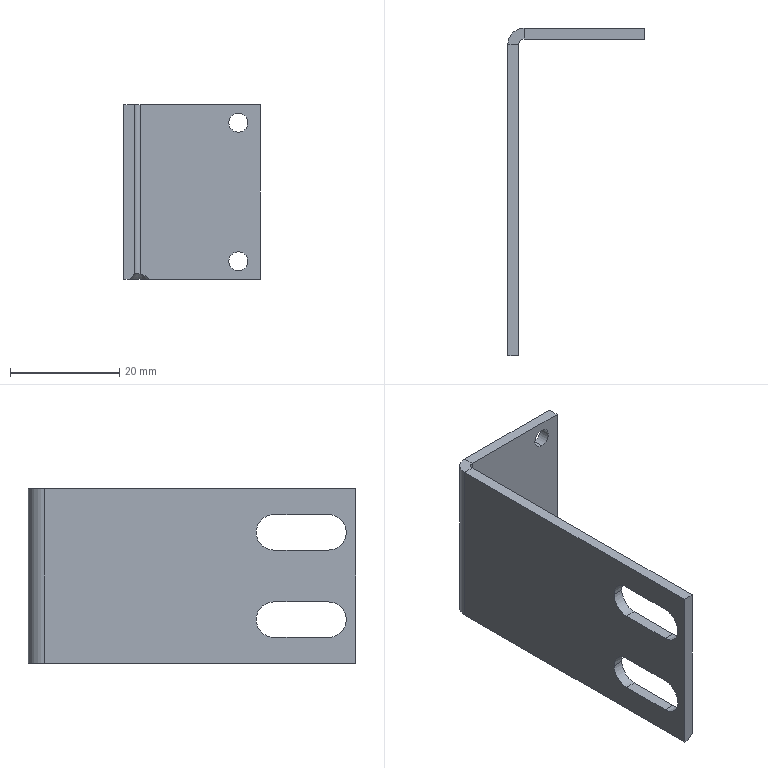Component | SolidWorks | 30-49A-1 | 1 solid | 30 faces | box 25 x 60 x 32 mm | volume 4796 mm3 | plane 17 | cylinder 12 | cone 1 | commonest cylinder face diameters 6.5 x6 3.5 x4 6 x1 2 x1
STEP:
#1=CARTESIAN_POINT('',(-33.473,1.02,11.797));
#2=VERTEX_POINT('',#1);
#3=CARTESIAN_POINT('',(-33.473,1.02,11.659));
#4=VERTEX_POINT('',#3);
#5=CARTESIAN_POINT('',(-33.473,1.02,11.728));
#6=DIRECTION('',(-0.,1.,-0.));
#7=DIRECTION('',(0.,0.,-1.));
#8=AXIS2_PLACEMENT_3D('',#5,#6,#7);
#9=CIRCLE('',#8,0.0689);
#10=EDGE_CURVE('',#2,#4,#9,.T.);
#11=ORIENTED_EDGE('',*,*,#10,.F.);
#12=CARTESIAN_POINT('',(-33.473,1.099,11.797));
#13=VERTEX_POINT('',#12);
#14=CARTESIAN_POINT('',(-33.473,1.099,11.797));
#15=DIRECTION('',(-0.,1.,-0.));
#16=VECTOR('',#15,39.37);
#17=LINE('',#14,#16);
#18=EDGE_CURVE('',#2,#13,#17,.T.);
#19=ORIENTED_EDGE('',*,*,#18,.T.);
#20=CARTESIAN_POINT('',(-33.473,1.099,11.659));
#21=VERTEX_POINT('',#20);
#22=CARTESIAN_POINT('',(-33.473,1.099,11.728));
#23=DIRECTION('',(-0.,1.,-0.));
#24=DIRECTION('',(0.,0.,-1.));
#25=AXIS2_PLACEMENT_3D('',#22,#23,#24);
#26=CIRCLE('',#25,0.0689);
#27=EDGE_CURVE('',#13,#21,#26,.T.);
#28=ORIENTED_EDGE('',*,*,#27,.T.);
#29=CARTESIAN_POINT('',(-33.473,1.099,11.659));
#30=DIRECTION('',(-0.,1.,-0.));
#31=VECTOR('',#30,39.37);
#32=LINE('',#29,#31);
#33=EDGE_CURVE('',#4,#21,#32,.T.);
#34=ORIENTED_EDGE('',*,*,#33,.F.);
#35=EDGE_LOOP('',(#11,#19,#28,#34));
#36=FACE_OUTER_BOUND('',#35,.T.);
#37=CARTESIAN_POINT('',(-33.473,1.099,11.728));
#38=DIRECTION('',(-0.,1.,-0.));
#39=DIRECTION('',(0.,0.,-1.));
#40=AXIS2_PLACEMENT_3D('',#37,#38,#39);
#41=CYLINDRICAL_SURFACE('',#40,0.0689);
#42=ADVANCED_FACE('',(#36),#41,.F.);
#43=CARTESIAN_POINT('',(-33.473,1.02,10.797));
#44=VERTEX_POINT('',#43);
#45=CARTESIAN_POINT('',(-33.473,1.02,10.659));
#46=VERTEX_POINT('',#45);
#47=CARTESIAN_POINT('',(-33.473,1.02,10.728));
#48=DIRECTION('',(-0.,1.,-0.));
#49=DIRECTION('',(0.,0.,-1.));
#50=AXIS2_PLACEMENT_3D('',#47,#48,#49);
#51=CIRCLE('',#50,0.0689);
#52=EDGE_CURVE('',#44,#46,#51,.T.);
#53=ORIENTED_EDGE('',*,*,#52,.F.);
#54=CARTESIAN_POINT('',(-33.473,1.099,10.797));
#55=VERTEX_POINT('',#54);
#56=CARTESIAN_POINT('',(-33.473,1.099,10.797));
#57=DIRECTION('',(-0.,1.,-0.));
#58=VECTOR('',#57,39.37);
#59=LINE('',#56,#58);
#60=EDGE_CURVE('',#44,#55,#59,.T.);
#61=ORIENTED_EDGE('',*,*,#60,.T.);
#62=CARTESIAN_POINT('',(-33.473,1.099,10.659));
#63=VERTEX_POINT('',#62);
#64=CARTESIAN_POINT('',(-33.473,1.099,10.728));
#65=DIRECTION('',(-0.,1.,-0.));
#66=DIRECTION('',(0.,0.,-1.));
#67=AXIS2_PLACEMENT_3D('',#64,#65,#66);
#68=CIRCLE('',#67,0.0689);
#69=EDGE_CURVE('',#55,#63,#68,.T.);
#70=ORIENTED_EDGE('',*,*,#69,.T.);
#71=CARTESIAN_POINT('',(-33.473,1.099,10.659));
#72=DIRECTION('',(-0.,1.,-0.));
#73=VECTOR('',#72,39.37);
#74=LINE('',#71,#73);
#75=EDGE_CURVE('',#46,#63,#74,.T.);
#76=ORIENTED_EDGE('',*,*,#75,.F.);
#77=EDGE_LOOP('',(#53,#61,#70,#76));
#78=FACE_OUTER_BOUND('',#77,.T.);
#79=CARTESIAN_POINT('',(-33.473,1.099,10.728));
#80=DIRECTION('',(-0.,1.,-0.));
#81=DIRECTION('',(0.,0.,-1.));
#82=AXIS2_PLACEMENT_3D('',#79,#80,#81);
#83=CYLINDRICAL_SURFACE('',#82,0.0689);
#84=ADVANCED_FACE('',(#78),#83,.F.);
#85=CARTESIAN_POINT('',(-34.221,-0.5449,11.543));
#86=VERTEX_POINT('',#85);
#87=CARTESIAN_POINT('',(-34.221,-0.6729,11.415));
#88=VERTEX_POINT('',#87);
#89=CARTESIAN_POINT('',(-34.221,-0.6729,11.543));
#90=DIRECTION('',(-1.,-0.,0.));
#91=DIRECTION('',(0.,1.,0.));
#92=AXIS2_PLACEMENT_3D('',#89,#90,#91);
#93=CIRCLE('',#92,0.128);
#94=EDGE_CURVE('',#86,#88,#93,.T.);
#95=ORIENTED_EDGE('',*,*,#94,.F.);
#96=CARTESIAN_POINT('',(-34.3,-0.5449,11.543));
#97=VERTEX_POINT('',#96);
#98=CARTESIAN_POINT('',(-33.315,-0.5449,11.543));
#99=DIRECTION('',(-1.,-0.,0.));
#100=VECTOR('',#99,39.37);
#101=LINE('',#98,#100);
#102=EDGE_CURVE('',#86,#97,#101,.T.);
#103=ORIENTED_EDGE('',*,*,#102,.T.);
#104=CARTESIAN_POINT('',(-34.3,-0.6729,11.415));
#105=VERTEX_POINT('',#104);
#106=CARTESIAN_POINT('',(-34.3,-0.6729,11.543));
#107=DIRECTION('',(-1.,-0.,0.));
#108=DIRECTION('',(0.,1.,0.));
#109=AXIS2_PLACEMENT_3D('',#106,#107,#108);
#110=CIRCLE('',#109,0.128);
#111=EDGE_CURVE('',#97,#105,#110,.T.);
#112=ORIENTED_EDGE('',*,*,#111,.T.);
#113=CARTESIAN_POINT('',(-33.315,-0.6729,11.415));
#114=DIRECTION('',(-1.,-0.,0.));
#115=VECTOR('',#114,39.37);
#116=LINE('',#113,#115);
#117=EDGE_CURVE('',#88,#105,#116,.T.);
#118=ORIENTED_EDGE('',*,*,#117,.F.);
#119=EDGE_LOOP('',(#95,#103,#112,#118));
#120=FACE_OUTER_BOUND('',#119,.T.);
#121=CARTESIAN_POINT('',(-33.315,-0.6729,11.543));
#122=DIRECTION('',(-1.,-0.,0.));
#123=DIRECTION('',(0.,1.,0.));
#124=AXIS2_PLACEMENT_3D('',#121,#122,#123);
#125=CYLINDRICAL_SURFACE('',#124,0.128);
#126=ADVANCED_FACE('',(#120),#125,.F.);
#127=CARTESIAN_POINT('',(-34.221,-0.5449,10.913));
#128=VERTEX_POINT('',#127);
#129=CARTESIAN_POINT('',(-34.221,-0.6729,10.785));
#130=VERTEX_POINT('',#129);
#131=CARTESIAN_POINT('',(-34.221,-0.6729,10.913));
#132=DIRECTION('',(-1.,-0.,0.));
#133=DIRECTION('',(0.,1.,0.));
#134=AXIS2_PLACEMENT_3D('',#131,#132,#133);
#135=CIRCLE('',#134,0.128);
#136=EDGE_CURVE('',#128,#130,#135,.T.);
#137=ORIENTED_EDGE('',*,*,#136,.F.);
#138=CARTESIAN_POINT('',(-34.3,-0.5449,10.913));
#139=VERTEX_POINT('',#138);
#140=CARTESIAN_POINT('',(-33.315,-0.5449,10.913));
#141=DIRECTION('',(-1.,-0.,0.));
#142=VECTOR('',#141,39.37);
#143=LINE('',#140,#142);
#144=EDGE_CURVE('',#128,#139,#143,.T.);
#145=ORIENTED_EDGE('',*,*,#144,.T.);
#146=CARTESIAN_POINT('',(-34.3,-0.6729,10.785));
#147=VERTEX_POINT('',#146);
#148=CARTESIAN_POINT('',(-34.3,-0.6729,10.913));
#149=DIRECTION('',(-1.,-0.,0.));
#150=DIRECTION('',(0.,-1.,0.));
#151=AXIS2_PLACEMENT_3D('',#148,#149,#150);
#152=CIRCLE('',#151,0.128);
#153=EDGE_CURVE('',#139,#147,#152,.T.);
#154=ORIENTED_EDGE('',*,*,#153,.T.);
#155=CARTESIAN_POINT('',(-33.315,-0.6729,10.785));
#156=DIRECTION('',(-1.,-0.,0.));
#157=VECTOR('',#156,39.37);
#158=LINE('',#155,#157);
#159=EDGE_CURVE('',#130,#147,#158,.T.);
#160=ORIENTED_EDGE('',*,*,#159,.F.);
#161=EDGE_LOOP('',(#137,#145,#154,#160));
#162=FACE_OUTER_BOUND('',#161,.T.);
#163=CARTESIAN_POINT('',(-33.315,-0.6729,10.913));
#164=DIRECTION('',(-1.,-0.,0.));
#165=DIRECTION('',(0.,1.,0.));
#166=AXIS2_PLACEMENT_3D('',#163,#164,#165);
#167=CYLINDRICAL_SURFACE('',#166,0.128);
#168=ADVANCED_FACE('',(#162),#167,.F.);
#169=CARTESIAN_POINT('',(-34.181,1.059,10.598));
#170=VERTEX_POINT('',#169);
#171=CARTESIAN_POINT('',(-34.181,1.099,10.598));
#172=VERTEX_POINT('',#171);
#173=CARTESIAN_POINT('',(-34.181,1.02,10.598));
#174=DIRECTION('',(-0.,1.,-0.));
#175=VECTOR('',#174,39.37);
#176=LINE('',#173,#175);
#177=EDGE_CURVE('',#170,#172,#176,.T.);
#178=ORIENTED_EDGE('',*,*,#177,.F.);
#179=CARTESIAN_POINT('',(-34.26,0.9806,10.598));
#180=VERTEX_POINT('',#179);
#181=CARTESIAN_POINT('',(-34.181,0.9806,10.598));
#182=DIRECTION('',(0.,0.,1.));
#183=DIRECTION('',(-1.,-0.,0.));
#184=AXIS2_PLACEMENT_3D('',#181,#182,#183);
#185=CIRCLE('',#184,0.07874);
#186=EDGE_CURVE('',#170,#180,#185,.T.);
#187=ORIENTED_EDGE('',*,*,#186,.T.);
#188=CARTESIAN_POINT('',(-34.3,0.9806,10.598));
#189=VERTEX_POINT('',#188);
#190=CARTESIAN_POINT('',(-34.3,0.9806,10.598));
#191=DIRECTION('',(1.,0.,-0.));
#192=VECTOR('',#191,39.37);
#193=LINE('',#190,#192);
#194=EDGE_CURVE('',#189,#180,#193,.T.);
#195=ORIENTED_EDGE('',*,*,#194,.F.);
#196=CARTESIAN_POINT('',(-34.181,0.9806,10.598));
#197=DIRECTION('',(0.,0.,1.));
#198=DIRECTION('',(-1.,-0.,0.));
#199=AXIS2_PLACEMENT_3D('',#196,#197,#198);
#200=CIRCLE('',#199,0.1181);
#201=EDGE_CURVE('',#172,#189,#200,.T.);
#202=ORIENTED_EDGE('',*,*,#201,.F.);
#203=EDGE_LOOP('',(#178,#187,#195,#202));
#204=FACE_OUTER_BOUND('',#203,.T.);
#205=CARTESIAN_POINT('',(-34.3,0.9806,10.598));
#206=DIRECTION('',(-0.,-0.,-1.));
#207=DIRECTION('',(-1.,-0.,0.));
#208=AXIS2_PLACEMENT_3D('',#205,#206,#207);
#209=PLANE('',#208);
#210=ADVANCED_FACE('',(#204),#209,.T.);
#211=ORIENTED_EDGE('',*,*,#194,.T.);
#212=CARTESIAN_POINT('',(-34.26,-1.263,10.598));
#213=VERTEX_POINT('',#212);
#214=CARTESIAN_POINT('',(-34.26,-1.263,10.598));
#215=DIRECTION('',(0.,-1.,0.));
#216=VECTOR('',#215,39.37);
#217=LINE('',#214,#216);
#218=EDGE_CURVE('',#180,#213,#217,.T.);
#219=ORIENTED_EDGE('',*,*,#218,.T.);
#220=CARTESIAN_POINT('',(-34.3,-1.263,10.598));
#221=VERTEX_POINT('',#220);
#222=CARTESIAN_POINT('',(-34.3,-1.263,10.598));
#223=DIRECTION('',(1.,0.,-0.));
#224=VECTOR('',#223,39.37);
#225=LINE('',#222,#224);
#226=EDGE_CURVE('',#221,#213,#225,.T.);
#227=ORIENTED_EDGE('',*,*,#226,.F.);
#228=CARTESIAN_POINT('',(-34.3,1.099,10.598));
#229=DIRECTION('',(0.,-1.,0.));
#230=VECTOR('',#229,39.37);
#231=LINE('',#228,#230);
#232=EDGE_CURVE('',#189,#221,#231,.T.);
#233=ORIENTED_EDGE('',*,*,#232,.F.);
#234=EDGE_LOOP('',(#211,#219,#227,#233));
#235=FACE_OUTER_BOUND('',#234,.T.);
#236=CARTESIAN_POINT('',(-34.181,1.02,10.598));
#237=DIRECTION('',(-0.,-0.,-1.));
#238=DIRECTION('',(-1.,-0.,0.));
#239=AXIS2_PLACEMENT_3D('',#236,#237,#238);
#240=PLANE('',#239);
#241=ADVANCED_FACE('',(#235),#240,.T.);
#242=CARTESIAN_POINT('',(-34.181,1.099,11.858));
#243=VERTEX_POINT('',#242);
#244=CARTESIAN_POINT('',(-34.181,1.02,11.858));
#245=VERTEX_POINT('',#244);
#246=CARTESIAN_POINT('',(-34.181,1.099,11.858));
#247=DIRECTION('',(0.,-1.,0.));
#248=VECTOR('',#247,39.37);
#249=LINE('',#246,#248);
#250=EDGE_CURVE('',#243,#245,#249,.T.);
#251=ORIENTED_EDGE('',*,*,#250,.F.);
#252=CARTESIAN_POINT('',(-34.3,0.9806,11.858));
#253=VERTEX_POINT('',#252);
#254=CARTESIAN_POINT('',(-34.181,0.9806,11.858));
#255=DIRECTION('',(0.,0.,1.));
#256=DIRECTION('',(-1.,-0.,0.));
#257=AXIS2_PLACEMENT_3D('',#254,#255,#256);
#258=CIRCLE('',#257,0.1181);
#259=EDGE_CURVE('',#243,#253,#258,.T.);
#260=ORIENTED_EDGE('',*,*,#259,.T.);
#261=CARTESIAN_POINT('',(-34.221,0.9806,11.858));
#262=VERTEX_POINT('',#261);
#263=CARTESIAN_POINT('',(-34.221,0.9806,11.858));
#264=DIRECTION('',(-1.,-0.,0.));
#265=VECTOR('',#264,39.37);
#266=LINE('',#263,#265);
#267=EDGE_CURVE('',#262,#253,#266,.T.);
#268=ORIENTED_EDGE('',*,*,#267,.F.);
#269=CARTESIAN_POINT('',(-34.181,0.9806,11.858));
#270=DIRECTION('',(0.,0.,1.));
#271=DIRECTION('',(-1.,-0.,0.));
#272=AXIS2_PLACEMENT_3D('',#269,#270,#271);
#273=CIRCLE('',#272,0.03937);
#274=EDGE_CURVE('',#245,#262,#273,.T.);
#275=ORIENTED_EDGE('',*,*,#274,.F.);
#276=EDGE_LOOP('',(#251,#260,#268,#275));
#277=FACE_OUTER_BOUND('',#276,.T.);
#278=CARTESIAN_POINT('',(-34.181,1.099,11.858));
#279=DIRECTION('',(0.,0.,1.));
#280=DIRECTION('',(1.,0.,-0.));
#281=AXIS2_PLACEMENT_3D('',#278,#279,#280);
#282=PLANE('',#281);
#283=ADVANCED_FACE('',(#277),#282,.T.);
#284=CARTESIAN_POINT('',(-33.315,1.099,11.858));
#285=VERTEX_POINT('',#284);
#286=CARTESIAN_POINT('',(-33.315,1.099,11.858));
#287=DIRECTION('',(-1.,-0.,0.));
#288=VECTOR('',#287,39.37);
#289=LINE('',#286,#288);
#290=EDGE_CURVE('',#285,#243,#289,.T.);
#291=ORIENTED_EDGE('',*,*,#290,.T.);
#292=ORIENTED_EDGE('',*,*,#250,.T.);
#293=CARTESIAN_POINT('',(-33.315,1.02,11.858));
#294=VERTEX_POINT('',#293);
#295=CARTESIAN_POINT('',(-33.315,1.02,11.858));
#296=DIRECTION('',(-1.,-0.,0.));
#297=VECTOR('',#296,39.37);
#298=LINE('',#295,#297);
#299=EDGE_CURVE('',#294,#245,#298,.T.);
#300=ORIENTED_EDGE('',*,*,#299,.F.);
#301=CARTESIAN_POINT('',(-33.315,1.02,11.858));
#302=DIRECTION('',(-0.,1.,-0.));
#303=VECTOR('',#302,39.37);
#304=LINE('',#301,#303);
#305=EDGE_CURVE('',#294,#285,#304,.T.);
#306=ORIENTED_EDGE('',*,*,#305,.T.);
#307=EDGE_LOOP('',(#291,#292,#300,#306));
#308=FACE_OUTER_BOUND('',#307,.T.);
#309=CARTESIAN_POINT('',(-34.221,0.9806,11.858));
#310=DIRECTION('',(0.,0.,1.));
#311=DIRECTION('',(1.,0.,-0.));
#312=AXIS2_PLACEMENT_3D('',#309,#310,#311);
#313=PLANE('',#312);
#314=ADVANCED_FACE('',(#308),#313,.T.);
#315=CARTESIAN_POINT('',(-34.221,-1.067,11.415));
#316=VERTEX_POINT('',#315);
#317=CARTESIAN_POINT('',(-34.221,1.099,11.415));
#318=DIRECTION('',(0.,-1.,0.));
#319=VECTOR('',#318,39.37);
#320=LINE('',#317,#319);
#321=EDGE_CURVE('',#88,#316,#320,.T.);
#322=ORIENTED_EDGE('',*,*,#321,.T.);
#323=CARTESIAN_POINT('',(-34.221,-1.067,11.671));
#324=VERTEX_POINT('',#323);
#325=CARTESIAN_POINT('',(-34.221,-1.067,11.543));
#326=DIRECTION('',(-1.,-0.,0.));
#327=DIRECTION('',(0.,1.,0.));
#328=AXIS2_PLACEMENT_3D('',#325,#326,#327);
#329=CIRCLE('',#328,0.128);
#330=EDGE_CURVE('',#316,#324,#329,.T.);
#331=ORIENTED_EDGE('',*,*,#330,.T.);
#332=CARTESIAN_POINT('',(-34.221,-0.6729,11.671));
#333=VERTEX_POINT('',#332);
#334=CARTESIAN_POINT('',(-34.221,1.099,11.671));
#335=DIRECTION('',(-0.,1.,-0.));
#336=VECTOR('',#335,39.37);
#337=LINE('',#334,#336);
#338=EDGE_CURVE('',#324,#333,#337,.T.);
#339=ORIENTED_EDGE('',*,*,#338,.T.);
#340=CARTESIAN_POINT('',(-34.221,-0.6729,11.543));
#341=DIRECTION('',(-1.,-0.,0.));
#342=DIRECTION('',(0.,1.,0.));
#343=AXIS2_PLACEMENT_3D('',#340,#341,#342);
#344=CIRCLE('',#343,0.128);
#345=EDGE_CURVE('',#333,#86,#344,.T.);
#346=ORIENTED_EDGE('',*,*,#345,.T.);
#347=ORIENTED_EDGE('',*,*,#94,.T.);
#348=EDGE_LOOP('',(#322,#331,#339,#346,#347));
#349=FACE_BOUND('',#348,.T.);
#350=CARTESIAN_POINT('',(-34.221,-1.067,11.041));
#351=VERTEX_POINT('',#350);
#352=CARTESIAN_POINT('',(-34.221,-0.6729,11.041));
#353=VERTEX_POINT('',#352);
#354=CARTESIAN_POINT('',(-34.221,1.099,11.041));
#355=DIRECTION('',(-0.,1.,-0.));
#356=VECTOR('',#355,39.37);
#357=LINE('',#354,#356);
#358=EDGE_CURVE('',#351,#353,#357,.T.);
#359=ORIENTED_EDGE('',*,*,#358,.T.);
#360=CARTESIAN_POINT('',(-34.221,-0.6729,10.913));
#361=DIRECTION('',(-1.,-0.,0.));
#362=DIRECTION('',(0.,1.,0.));
#363=AXIS2_PLACEMENT_3D('',#360,#361,#362);
#364=CIRCLE('',#363,0.128);
#365=EDGE_CURVE('',#353,#128,#364,.T.);
#366=ORIENTED_EDGE('',*,*,#365,.T.);
#367=ORIENTED_EDGE('',*,*,#136,.T.);
#368=CARTESIAN_POINT('',(-34.221,-1.067,10.785));
#369=VERTEX_POINT('',#368);
#370=CARTESIAN_POINT('',(-34.221,1.099,10.785));
#371=DIRECTION('',(0.,-1.,0.));
#372=VECTOR('',#371,39.37);
#373=LINE('',#370,#372);
#374=EDGE_CURVE('',#130,#369,#373,.T.);
#375=ORIENTED_EDGE('',*,*,#374,.T.);
#376=CARTESIAN_POINT('',(-34.221,-1.067,10.913));
#377=DIRECTION('',(-1.,-0.,0.));
#378=DIRECTION('',(0.,1.,0.));
#379=AXIS2_PLACEMENT_3D('',#376,#377,#378);
#380=CIRCLE('',#379,0.128);
#381=EDGE_CURVE('',#369,#351,#380,.T.);
#382=ORIENTED_EDGE('',*,*,#381,.T.);
#383=EDGE_LOOP('',(#359,#366,#367,#375,#382));
#384=FACE_BOUND('',#383,.T.);
#385=CARTESIAN_POINT('',(-34.221,-1.263,10.637));
#386=VERTEX_POINT('',#385);
#387=CARTESIAN_POINT('',(-34.221,-1.263,11.858));
#388=VERTEX_POINT('',#387);
#389=CARTESIAN_POINT('',(-34.221,-1.263,10.598));
#390=DIRECTION('',(0.,0.,1.));
#391=VECTOR('',#390,39.37);
#392=LINE('',#389,#391);
#393=EDGE_CURVE('',#386,#388,#392,.T.);
#394=ORIENTED_EDGE('',*,*,#393,.F.);
#395=CARTESIAN_POINT('',(-34.221,0.9806,10.637));
#396=VERTEX_POINT('',#395);
#397=CARTESIAN_POINT('',(-34.221,0.9806,10.637));
#398=DIRECTION('',(-0.,1.,-0.));
#399=VECTOR('',#398,39.37);
#400=LINE('',#397,#399);
#401=EDGE_CURVE('',#386,#396,#400,.T.);
#402=ORIENTED_EDGE('',*,*,#401,.T.);
#403=CARTESIAN_POINT('',(-34.221,0.9806,10.598));
#404=DIRECTION('',(0.,0.,1.));
#405=VECTOR('',#404,39.37);
#406=LINE('',#403,#405);
#407=EDGE_CURVE('',#396,#262,#406,.T.);
#408=ORIENTED_EDGE('',*,*,#407,.T.);
#409=CARTESIAN_POINT('',(-34.221,1.099,11.858));
#410=DIRECTION('',(0.,-1.,0.));
#411=VECTOR('',#410,39.37);
#412=LINE('',#409,#411);
#413=EDGE_CURVE('',#262,#388,#412,.T.);
#414=ORIENTED_EDGE('',*,*,#413,.T.);
#415=EDGE_LOOP('',(#394,#402,#408,#414));
#416=FACE_OUTER_BOUND('',#415,.T.);
#417=CARTESIAN_POINT('',(-34.221,1.099,10.598));
#418=DIRECTION('',(-1.,-0.,0.));
#419=DIRECTION('',(-0.,1.,-0.));
#420=AXIS2_PLACEMENT_3D('',#417,#418,#419);
#421=PLANE('',#420);
#422=ADVANCED_FACE('',(#349,#384,#416),#421,.F.);
#423=ORIENTED_EDGE('',*,*,#226,.T.);
#424=CARTESIAN_POINT('',(-34.28,-1.263,10.578));
#425=DIRECTION('',(0.7071,0.,0.7071));
#426=VECTOR('',#425,39.37);
#427=LINE('',#424,#426);
#428=EDGE_CURVE('',#213,#386,#427,.T.);
#429=ORIENTED_EDGE('',*,*,#428,.T.);
#430=ORIENTED_EDGE('',*,*,#393,.T.);
#431=CARTESIAN_POINT('',(-34.3,-1.263,11.858));
#432=VERTEX_POINT('',#431);
#433=CARTESIAN_POINT('',(-34.3,-1.263,11.858));
#434=DIRECTION('',(1.,0.,-0.));
#435=VECTOR('',#434,39.37);
#436=LINE('',#433,#435);
#437=EDGE_CURVE('',#432,#388,#436,.T.);
#438=ORIENTED_EDGE('',*,*,#437,.F.);
#439=CARTESIAN_POINT('',(-34.3,-1.263,10.598));
#440=DIRECTION('',(0.,0.,1.));
#441=VECTOR('',#440,39.37);
#442=LINE('',#439,#441);
#443=EDGE_CURVE('',#221,#432,#442,.T.);
#444=ORIENTED_EDGE('',*,*,#443,.F.);
#445=EDGE_LOOP('',(#423,#429,#430,#438,#444));
#446=FACE_OUTER_BOUND('',#445,.T.);
#447=CARTESIAN_POINT('',(-34.3,-1.263,10.598));
#448=DIRECTION('',(0.,-1.,0.));
#449=DIRECTION('',(0.,0.,1.));
#450=AXIS2_PLACEMENT_3D('',#447,#448,#449);
#451=PLANE('',#450);
#452=ADVANCED_FACE('',(#446),#451,.T.);
#453=CARTESIAN_POINT('',(-34.3,-1.067,11.415));
#454=VERTEX_POINT('',#453);
#455=CARTESIAN_POINT('',(-34.3,-1.067,11.671));
#456=VERTEX_POINT('',#455);
#457=CARTESIAN_POINT('',(-34.3,-1.067,11.543));
#458=DIRECTION('',(-1.,-0.,0.));
#459=DIRECTION('',(0.,-1.,0.));
#460=AXIS2_PLACEMENT_3D('',#457,#458,#459);
#461=CIRCLE('',#460,0.128);
#462=EDGE_CURVE('',#454,#456,#461,.T.);
#463=ORIENTED_EDGE('',*,*,#462,.F.);
#464=CARTESIAN_POINT('',(-34.3,-0.6729,11.415));
#465=DIRECTION('',(0.,-1.,0.));
#466=VECTOR('',#465,39.37);
#467=LINE('',#464,#466);
#468=EDGE_CURVE('',#105,#454,#467,.T.);
#469=ORIENTED_EDGE('',*,*,#468,.F.);
#470=ORIENTED_EDGE('',*,*,#111,.F.);
#471=CARTESIAN_POINT('',(-34.3,-0.6729,11.671));
#472=VERTEX_POINT('',#471);
#473=CARTESIAN_POINT('',(-34.3,-0.6729,11.543));
#474=DIRECTION('',(-1.,-0.,0.));
#475=DIRECTION('',(0.,1.,0.));
#476=AXIS2_PLACEMENT_3D('',#473,#474,#475);
#477=CIRCLE('',#476,0.128);
#478=EDGE_CURVE('',#472,#97,#477,.T.);
#479=ORIENTED_EDGE('',*,*,#478,.F.);
#480=CARTESIAN_POINT('',(-34.3,-0.6729,11.671));
#481=DIRECTION('',(-0.,1.,-0.));
#482=VECTOR('',#481,39.37);
#483=LINE('',#480,#482);
#484=EDGE_CURVE('',#456,#472,#483,.T.);
#485=ORIENTED_EDGE('',*,*,#484,.F.);
#486=EDGE_LOOP('',(#463,#469,#470,#479,#485));
#487=FACE_BOUND('',#486,.T.);
#488=CARTESIAN_POINT('',(-34.3,-0.6729,11.041));
#489=VERTEX_POINT('',#488);
#490=CARTESIAN_POINT('',(-34.3,-0.6729,10.913));
#491=DIRECTION('',(-1.,-0.,0.));
#492=DIRECTION('',(0.,-1.,0.));
#493=AXIS2_PLACEMENT_3D('',#490,#491,#492);
#494=CIRCLE('',#493,0.128);
#495=EDGE_CURVE('',#489,#139,#494,.T.);
#496=ORIENTED_EDGE('',*,*,#495,.F.);
#497=CARTESIAN_POINT('',(-34.3,-1.067,11.041));
#498=VERTEX_POINT('',#497);
#499=CARTESIAN_POINT('',(-34.3,-0.6729,11.041));
#500=DIRECTION('',(-0.,1.,-0.));
#501=VECTOR('',#500,39.37);
#502=LINE('',#499,#501);
#503=EDGE_CURVE('',#498,#489,#502,.T.);
#504=ORIENTED_EDGE('',*,*,#503,.F.);
#505=CARTESIAN_POINT('',(-34.3,-1.067,10.785));
#506=VERTEX_POINT('',#505);
#507=CARTESIAN_POINT('',(-34.3,-1.067,10.913));
#508=DIRECTION('',(-1.,-0.,0.));
#509=DIRECTION('',(0.,1.,0.));
#510=AXIS2_PLACEMENT_3D('',#507,#508,#509);
#511=CIRCLE('',#510,0.128);
#512=EDGE_CURVE('',#506,#498,#511,.T.);
#513=ORIENTED_EDGE('',*,*,#512,.F.);
#514=CARTESIAN_POINT('',(-34.3,-0.6729,10.785));
#515=DIRECTION('',(0.,-1.,0.));
#516=VECTOR('',#515,39.37);
#517=LINE('',#514,#516);
#518=EDGE_CURVE('',#147,#506,#517,.T.);
#519=ORIENTED_EDGE('',*,*,#518,.F.);
#520=ORIENTED_EDGE('',*,*,#153,.F.);
#521=EDGE_LOOP('',(#496,#504,#513,#519,#520));
#522=FACE_BOUND('',#521,.T.);
#523=CARTESIAN_POINT('',(-34.3,1.099,11.858));
#524=DIRECTION('',(0.,-1.,0.));
#525=VECTOR('',#524,39.37);
#526=LINE('',#523,#525);
#527=EDGE_CURVE('',#253,#432,#526,.T.);
#528=ORIENTED_EDGE('',*,*,#527,.F.);
#529=CARTESIAN_POINT('',(-34.3,0.9806,10.598));
#530=DIRECTION('',(0.,0.,1.));
#531=VECTOR('',#530,39.37);
#532=LINE('',#529,#531);
#533=EDGE_CURVE('',#189,#253,#532,.T.);
#534=ORIENTED_EDGE('',*,*,#533,.F.);
#535=ORIENTED_EDGE('',*,*,#232,.T.);
#536=ORIENTED_EDGE('',*,*,#443,.T.);
#537=EDGE_LOOP('',(#528,#534,#535,#536));
#538=FACE_OUTER_BOUND('',#537,.T.);
#539=CARTESIAN_POINT('',(-34.3,1.099,10.598));
#540=DIRECTION('',(-1.,-0.,0.));
#541=DIRECTION('',(-0.,1.,-0.));
#542=AXIS2_PLACEMENT_3D('',#539,#540,#541);
#543=PLANE('',#542);
#544=ADVANCED_FACE('',(#487,#522,#538),#543,.T.);
#545=ORIENTED_EDGE('',*,*,#259,.F.);
#546=CARTESIAN_POINT('',(-34.181,1.099,10.598));
#547=DIRECTION('',(0.,0.,1.));
#548=VECTOR('',#547,39.37);
#549=LINE('',#546,#548);
#550=EDGE_CURVE('',#172,#243,#549,.T.);
#551=ORIENTED_EDGE('',*,*,#550,.F.);
#552=ORIENTED_EDGE('',*,*,#201,.T.);
#553=ORIENTED_EDGE('',*,*,#533,.T.);
#554=EDGE_LOOP('',(#545,#551,#552,#553));
#555=FACE_OUTER_BOUND('',#554,.T.);
#556=CARTESIAN_POINT('',(-34.181,0.9806,10.598));
#557=DIRECTION('',(0.,0.,1.));
#558=DIRECTION('',(1.,0.,0.));
#559=AXIS2_PLACEMENT_3D('',#556,#557,#558);
#560=CYLINDRICAL_SURFACE('',#559,0.1181);
#561=ADVANCED_FACE('',(#555),#560,.T.);
#562=CARTESIAN_POINT('',(-33.473,1.099,11.728));
#563=DIRECTION('',(-0.,1.,-0.));
#564=DIRECTION('',(0.,0.,-1.));
#565=AXIS2_PLACEMENT_3D('',#562,#563,#564);
#566=CIRCLE('',#565,0.0689);
#567=EDGE_CURVE('',#21,#13,#566,.T.);
#568=ORIENTED_EDGE('',*,*,#567,.F.);
#569=ORIENTED_EDGE('',*,*,#27,.F.);
#570=EDGE_LOOP('',(#568,#569));
#571=FACE_BOUND('',#570,.T.);
#572=CARTESIAN_POINT('',(-33.473,1.099,10.728));
#573=DIRECTION('',(-0.,1.,-0.));
#574=DIRECTION('',(0.,0.,-1.));
#575=AXIS2_PLACEMENT_3D('',#572,#573,#574);
#576=CIRCLE('',#575,0.0689);
#577=EDGE_CURVE('',#63,#55,#576,.T.);
#578=ORIENTED_EDGE('',*,*,#577,.F.);
#579=ORIENTED_EDGE('',*,*,#69,.F.);
#580=EDGE_LOOP('',(#578,#579));
#581=FACE_BOUND('',#580,.T.);
#582=ORIENTED_EDGE('',*,*,#290,.F.);
#583=CARTESIAN_POINT('',(-33.315,1.099,10.598));
#584=VERTEX_POINT('',#583);
#585=CARTESIAN_POINT('',(-33.315,1.099,10.598));
#586=DIRECTION('',(0.,0.,1.));
#587=VECTOR('',#586,39.37);
#588=LINE('',#585,#587);
#589=EDGE_CURVE('',#584,#285,#588,.T.);
#590=ORIENTED_EDGE('',*,*,#589,.F.);
#591=CARTESIAN_POINT('',(-33.315,1.099,10.598));
#592=DIRECTION('',(-1.,-0.,0.));
#593=VECTOR('',#592,39.37);
#594=LINE('',#591,#593);
#595=EDGE_CURVE('',#584,#172,#594,.T.);
#596=ORIENTED_EDGE('',*,*,#595,.T.);
#597=ORIENTED_EDGE('',*,*,#550,.T.);
#598=EDGE_LOOP('',(#582,#590,#596,#597));
#599=FACE_OUTER_BOUND('',#598,.T.);
#600=CARTESIAN_POINT('',(-33.315,1.099,10.598));
#601=DIRECTION('',(-0.,1.,-0.));
#602=DIRECTION('',(-0.,-0.,-1.));
#603=AXIS2_PLACEMENT_3D('',#600,#601,#602);
#604=PLANE('',#603);
#605=ADVANCED_FACE('',(#571,#581,#599),#604,.T.);
#606=ORIENTED_EDGE('',*,*,#305,.F.);
#607=CARTESIAN_POINT('',(-33.315,1.02,10.598));
#608=VERTEX_POINT('',#607);
#609=CARTESIAN_POINT('',(-33.315,1.02,10.598));
#610=DIRECTION('',(0.,0.,1.));
#611=VECTOR('',#610,39.37);
#612=LINE('',#609,#611);
#613=EDGE_CURVE('',#608,#294,#612,.T.);
#614=ORIENTED_EDGE('',*,*,#613,.F.);
#615=CARTESIAN_POINT('',(-33.315,1.02,10.598));
#616=DIRECTION('',(-0.,1.,-0.));
#617=VECTOR('',#616,39.37);
#618=LINE('',#615,#617);
#619=EDGE_CURVE('',#608,#584,#618,.T.);
#620=ORIENTED_EDGE('',*,*,#619,.T.);
#621=ORIENTED_EDGE('',*,*,#589,.T.);
#622=EDGE_LOOP('',(#606,#614,#620,#621));
#623=FACE_OUTER_BOUND('',#622,.T.);
#624=CARTESIAN_POINT('',(-33.315,1.02,10.598));
#625=DIRECTION('',(1.,0.,-0.));
#626=DIRECTION('',(-0.,-0.,-1.));
#627=AXIS2_PLACEMENT_3D('',#624,#625,#626);
#628=PLANE('',#627);
#629=ADVANCED_FACE('',(#623),#628,.T.);
#630=CARTESIAN_POINT('',(-33.473,1.02,11.728));
#631=DIRECTION('',(-0.,1.,-0.));
#632=DIRECTION('',(0.,0.,-1.));
#633=AXIS2_PLACEMENT_3D('',#630,#631,#632);
#634=CIRCLE('',#633,0.0689);
#635=EDGE_CURVE('',#4,#2,#634,.T.);
#636=ORIENTED_EDGE('',*,*,#635,.T.);
#637=ORIENTED_EDGE('',*,*,#10,.T.);
#638=EDGE_LOOP('',(#636,#637));
#639=FACE_BOUND('',#638,.T.);
#640=CARTESIAN_POINT('',(-33.473,1.02,10.728));
#641=DIRECTION('',(-0.,1.,-0.));
#642=DIRECTION('',(0.,0.,-1.));
#643=AXIS2_PLACEMENT_3D('',#640,#641,#642);
#644=CIRCLE('',#643,0.0689);
#645=EDGE_CURVE('',#46,#44,#644,.T.);
#646=ORIENTED_EDGE('',*,*,#645,.T.);
#647=ORIENTED_EDGE('',*,*,#52,.T.);
#648=EDGE_LOOP('',(#646,#647));
#649=FACE_BOUND('',#648,.T.);
#650=CARTESIAN_POINT('',(-34.181,1.02,10.637));
#651=VERTEX_POINT('',#650);
#652=CARTESIAN_POINT('',(-34.181,1.02,10.598));
#653=DIRECTION('',(0.,0.,1.));
#654=VECTOR('',#653,39.37);
#655=LINE('',#652,#654);
#656=EDGE_CURVE('',#651,#245,#655,.T.);
#657=ORIENTED_EDGE('',*,*,#656,.F.);
#658=CARTESIAN_POINT('',(-34.113,1.02,10.598));
#659=VERTEX_POINT('',#658);
#660=CARTESIAN_POINT('',(-34.181,1.02,10.637));
#661=CARTESIAN_POINT('',(-34.175,1.02,10.637));
#662=CARTESIAN_POINT('',(-34.168,1.02,10.635));
#663=CARTESIAN_POINT('',(-34.156,1.02,10.63));
#664=CARTESIAN_POINT('',(-34.15,1.02,10.627));
#665=CARTESIAN_POINT('',(-34.134,1.02,10.615));
#666=CARTESIAN_POINT('',(-34.123,1.02,10.607));
#667=CARTESIAN_POINT('',(-34.113,1.02,10.598));
#668=B_SPLINE_CURVE_WITH_KNOTS('',3,(#660,#661,#662,#663,#664,#665,#666,#667),.UNSPECIFIED.,.F.,.F.,(4,2,2,4),(0.,0.0005094,0.001019,0.002038),.UNSPECIFIED.);
#669=EDGE_CURVE('',#651,#659,#668,.T.);
#670=ORIENTED_EDGE('',*,*,#669,.T.);
#671=CARTESIAN_POINT('',(-33.315,1.02,10.598));
#672=DIRECTION('',(-1.,-0.,0.));
#673=VECTOR('',#672,39.37);
#674=LINE('',#671,#673);
#675=EDGE_CURVE('',#608,#659,#674,.T.);
#676=ORIENTED_EDGE('',*,*,#675,.F.);
#677=ORIENTED_EDGE('',*,*,#613,.T.);
#678=ORIENTED_EDGE('',*,*,#299,.T.);
#679=EDGE_LOOP('',(#657,#670,#676,#677,#678));
#680=FACE_OUTER_BOUND('',#679,.T.);
#681=CARTESIAN_POINT('',(-33.315,1.02,10.598));
#682=DIRECTION('',(-0.,1.,-0.));
#683=DIRECTION('',(-0.,-0.,-1.));
#684=AXIS2_PLACEMENT_3D('',#681,#682,#683);
#685=PLANE('',#684);
#686=ADVANCED_FACE('',(#639,#649,#680),#685,.F.);
#687=ORIENTED_EDGE('',*,*,#407,.F.);
#688=CARTESIAN_POINT('',(-34.181,0.9806,10.637));
#689=DIRECTION('',(-0.,-0.,-1.));
#690=DIRECTION('',(-1.,-0.,0.));
#691=AXIS2_PLACEMENT_3D('',#688,#689,#690);
#692=CIRCLE('',#691,0.03937);
#693=EDGE_CURVE('',#396,#651,#692,.T.);
#694=ORIENTED_EDGE('',*,*,#693,.T.);
#695=ORIENTED_EDGE('',*,*,#656,.T.);
#696=ORIENTED_EDGE('',*,*,#274,.T.);
#697=EDGE_LOOP('',(#687,#694,#695,#696));
#698=FACE_OUTER_BOUND('',#697,.T.);
#699=CARTESIAN_POINT('',(-34.181,0.9806,10.598));
#700=DIRECTION('',(0.,0.,1.));
#701=DIRECTION('',(1.,0.,0.));
#702=AXIS2_PLACEMENT_3D('',#699,#700,#701);
#703=CYLINDRICAL_SURFACE('',#702,0.03937);
#704=ADVANCED_FACE('',(#698),#703,.F.);
#705=ORIENTED_EDGE('',*,*,#675,.T.);
#706=CARTESIAN_POINT('',(-34.181,0.9806,10.598));
#707=DIRECTION('',(0.,0.,1.));
#708=DIRECTION('',(-1.,-0.,0.));
#709=AXIS2_PLACEMENT_3D('',#706,#707,#708);
#710=CIRCLE('',#709,0.07874);
#711=EDGE_CURVE('',#659,#170,#710,.T.);
#712=ORIENTED_EDGE('',*,*,#711,.T.);
#713=ORIENTED_EDGE('',*,*,#177,.T.);
#714=ORIENTED_EDGE('',*,*,#595,.F.);
#715=ORIENTED_EDGE('',*,*,#619,.F.);
#716=EDGE_LOOP('',(#705,#712,#713,#714,#715));
#717=FACE_OUTER_BOUND('',#716,.T.);
#718=CARTESIAN_POINT('',(-34.181,0.9806,10.598));
#719=DIRECTION('',(-0.,-0.,-1.));
#720=DIRECTION('',(-1.,-0.,0.));
#721=AXIS2_PLACEMENT_3D('',#718,#719,#720);
#722=PLANE('',#721);
#723=ADVANCED_FACE('',(#717),#722,.T.);
#724=ORIENTED_EDGE('',*,*,#413,.F.);
#725=ORIENTED_EDGE('',*,*,#267,.T.);
#726=ORIENTED_EDGE('',*,*,#527,.T.);
#727=ORIENTED_EDGE('',*,*,#437,.T.);
#728=EDGE_LOOP('',(#724,#725,#726,#727));
#729=FACE_OUTER_BOUND('',#728,.T.);
#730=CARTESIAN_POINT('',(-34.181,0.9806,11.858));
#731=DIRECTION('',(-0.,-0.,-1.));
#732=DIRECTION('',(-1.,-0.,0.));
#733=AXIS2_PLACEMENT_3D('',#730,#731,#732);
#734=PLANE('',#733);
#735=ADVANCED_FACE('',(#729),#734,.F.);
#736=ORIENTED_EDGE('',*,*,#144,.F.);
#737=ORIENTED_EDGE('',*,*,#365,.F.);
#738=CARTESIAN_POINT('',(-33.315,-0.6729,11.041));
#739=DIRECTION('',(-1.,-0.,0.));
#740=VECTOR('',#739,39.37);
#741=LINE('',#738,#740);
#742=EDGE_CURVE('',#353,#489,#741,.T.);
#743=ORIENTED_EDGE('',*,*,#742,.T.);
#744=ORIENTED_EDGE('',*,*,#495,.T.);
#745=EDGE_LOOP('',(#736,#737,#743,#744));
#746=FACE_OUTER_BOUND('',#745,.T.);
#747=CARTESIAN_POINT('',(-33.315,-0.6729,10.913));
#748=DIRECTION('',(-1.,-0.,0.));
#749=DIRECTION('',(0.,1.,0.));
#750=AXIS2_PLACEMENT_3D('',#747,#748,#749);
#751=CYLINDRICAL_SURFACE('',#750,0.128);
#752=ADVANCED_FACE('',(#746),#751,.F.);
#753=CARTESIAN_POINT('',(-33.315,-1.067,11.041));
#754=DIRECTION('',(-1.,-0.,0.));
#755=VECTOR('',#754,39.37);
#756=LINE('',#753,#755);
#757=EDGE_CURVE('',#351,#498,#756,.T.);
#758=ORIENTED_EDGE('',*,*,#757,.T.);
#759=ORIENTED_EDGE('',*,*,#503,.T.);
#760=ORIENTED_EDGE('',*,*,#742,.F.);
#761=ORIENTED_EDGE('',*,*,#358,.F.);
#762=EDGE_LOOP('',(#758,#759,#760,#761));
#763=FACE_OUTER_BOUND('',#762,.T.);
#764=CARTESIAN_POINT('',(-33.315,-0.6729,11.041));
#765=DIRECTION('',(0.,0.,1.));
#766=DIRECTION('',(1.,0.,-0.));
#767=AXIS2_PLACEMENT_3D('',#764,#765,#766);
#768=PLANE('',#767);
#769=ADVANCED_FACE('',(#763),#768,.F.);
#770=CARTESIAN_POINT('',(-33.315,-1.067,10.785));
#771=DIRECTION('',(-1.,-0.,0.));
#772=VECTOR('',#771,39.37);
#773=LINE('',#770,#772);
#774=EDGE_CURVE('',#369,#506,#773,.T.);
#775=ORIENTED_EDGE('',*,*,#774,.T.);
#776=ORIENTED_EDGE('',*,*,#512,.T.);
#777=ORIENTED_EDGE('',*,*,#757,.F.);
#778=ORIENTED_EDGE('',*,*,#381,.F.);
#779=EDGE_LOOP('',(#775,#776,#777,#778));
#780=FACE_OUTER_BOUND('',#779,.T.);
#781=CARTESIAN_POINT('',(-33.315,-1.067,10.913));
#782=DIRECTION('',(-1.,-0.,0.));
#783=DIRECTION('',(0.,1.,0.));
#784=AXIS2_PLACEMENT_3D('',#781,#782,#783);
#785=CYLINDRICAL_SURFACE('',#784,0.128);
#786=ADVANCED_FACE('',(#780),#785,.F.);
#787=ORIENTED_EDGE('',*,*,#159,.T.);
#788=ORIENTED_EDGE('',*,*,#518,.T.);
#789=ORIENTED_EDGE('',*,*,#774,.F.);
#790=ORIENTED_EDGE('',*,*,#374,.F.);
#791=EDGE_LOOP('',(#787,#788,#789,#790));
#792=FACE_OUTER_BOUND('',#791,.T.);
#793=CARTESIAN_POINT('',(-33.315,-0.6729,10.785));
#794=DIRECTION('',(-0.,-0.,-1.));
#795=DIRECTION('',(-1.,-0.,0.));
#796=AXIS2_PLACEMENT_3D('',#793,#794,#795);
#797=PLANE('',#796);
#798=ADVANCED_FACE('',(#792),#797,.F.);
#799=CARTESIAN_POINT('',(-33.315,-1.067,11.415));
#800=DIRECTION('',(-1.,-0.,0.));
#801=VECTOR('',#800,39.37);
#802=LINE('',#799,#801);
#803=EDGE_CURVE('',#316,#454,#802,.T.);
#804=ORIENTED_EDGE('',*,*,#803,.T.);
#805=ORIENTED_EDGE('',*,*,#462,.T.);
#806=CARTESIAN_POINT('',(-33.315,-1.067,11.671));
#807=DIRECTION('',(-1.,-0.,0.));
#808=VECTOR('',#807,39.37);
#809=LINE('',#806,#808);
#810=EDGE_CURVE('',#324,#456,#809,.T.);
#811=ORIENTED_EDGE('',*,*,#810,.F.);
#812=ORIENTED_EDGE('',*,*,#330,.F.);
#813=EDGE_LOOP('',(#804,#805,#811,#812));
#814=FACE_OUTER_BOUND('',#813,.T.);
#815=CARTESIAN_POINT('',(-33.315,-1.067,11.543));
#816=DIRECTION('',(-1.,-0.,0.));
#817=DIRECTION('',(0.,1.,0.));
#818=AXIS2_PLACEMENT_3D('',#815,#816,#817);
#819=CYLINDRICAL_SURFACE('',#818,0.128);
#820=ADVANCED_FACE('',(#814),#819,.F.);
#821=ORIENTED_EDGE('',*,*,#117,.T.);
#822=ORIENTED_EDGE('',*,*,#468,.T.);
#823=ORIENTED_EDGE('',*,*,#803,.F.);
#824=ORIENTED_EDGE('',*,*,#321,.F.);
#825=EDGE_LOOP('',(#821,#822,#823,#824));
#826=FACE_OUTER_BOUND('',#825,.T.);
#827=CARTESIAN_POINT('',(-33.315,-0.6729,11.415));
#828=DIRECTION('',(-0.,-0.,-1.));
#829=DIRECTION('',(-1.,-0.,0.));
#830=AXIS2_PLACEMENT_3D('',#827,#828,#829);
#831=PLANE('',#830);
#832=ADVANCED_FACE('',(#826),#831,.F.);
#833=ORIENTED_EDGE('',*,*,#102,.F.);
#834=ORIENTED_EDGE('',*,*,#345,.F.);
#835=CARTESIAN_POINT('',(-33.315,-0.6729,11.671));
#836=DIRECTION('',(-1.,-0.,0.));
#837=VECTOR('',#836,39.37);
#838=LINE('',#835,#837);
#839=EDGE_CURVE('',#333,#472,#838,.T.);
#840=ORIENTED_EDGE('',*,*,#839,.T.);
#841=ORIENTED_EDGE('',*,*,#478,.T.);
#842=EDGE_LOOP('',(#833,#834,#840,#841));
#843=FACE_OUTER_BOUND('',#842,.T.);
#844=CARTESIAN_POINT('',(-33.315,-0.6729,11.543));
#845=DIRECTION('',(-1.,-0.,0.));
#846=DIRECTION('',(0.,1.,0.));
#847=AXIS2_PLACEMENT_3D('',#844,#845,#846);
#848=CYLINDRICAL_SURFACE('',#847,0.128);
#849=ADVANCED_FACE('',(#843),#848,.F.);
#850=ORIENTED_EDGE('',*,*,#810,.T.);
#851=ORIENTED_EDGE('',*,*,#484,.T.);
#852=ORIENTED_EDGE('',*,*,#839,.F.);
#853=ORIENTED_EDGE('',*,*,#338,.F.);
#854=EDGE_LOOP('',(#850,#851,#852,#853));
#855=FACE_OUTER_BOUND('',#854,.T.);
#856=CARTESIAN_POINT('',(-33.315,-0.6729,11.671));
#857=DIRECTION('',(0.,0.,1.));
#858=DIRECTION('',(1.,0.,-0.));
#859=AXIS2_PLACEMENT_3D('',#856,#857,#858);
#860=PLANE('',#859);
#861=ADVANCED_FACE('',(#855),#860,.F.);
#862=ORIENTED_EDGE('',*,*,#60,.F.);
#863=ORIENTED_EDGE('',*,*,#645,.F.);
#864=ORIENTED_EDGE('',*,*,#75,.T.);
#865=ORIENTED_EDGE('',*,*,#577,.T.);
#866=EDGE_LOOP('',(#862,#863,#864,#865));
#867=FACE_OUTER_BOUND('',#866,.T.);
#868=CARTESIAN_POINT('',(-33.473,1.099,10.728));
#869=DIRECTION('',(-0.,1.,-0.));
#870=DIRECTION('',(0.,0.,-1.));
#871=AXIS2_PLACEMENT_3D('',#868,#869,#870);
#872=CYLINDRICAL_SURFACE('',#871,0.0689);
#873=ADVANCED_FACE('',(#867),#872,.F.);
#874=ORIENTED_EDGE('',*,*,#18,.F.);
#875=ORIENTED_EDGE('',*,*,#635,.F.);
#876=ORIENTED_EDGE('',*,*,#33,.T.);
#877=ORIENTED_EDGE('',*,*,#567,.T.);
#878=EDGE_LOOP('',(#874,#875,#876,#877));
#879=FACE_OUTER_BOUND('',#878,.T.);
#880=CARTESIAN_POINT('',(-33.473,1.099,11.728));
#881=DIRECTION('',(-0.,1.,-0.));
#882=DIRECTION('',(0.,0.,-1.));
#883=AXIS2_PLACEMENT_3D('',#880,#881,#882);
#884=CYLINDRICAL_SURFACE('',#883,0.0689);
#885=ADVANCED_FACE('',(#879),#884,.F.);
#886=ORIENTED_EDGE('',*,*,#428,.F.);
#887=ORIENTED_EDGE('',*,*,#218,.F.);
#888=CARTESIAN_POINT('',(-34.221,0.9806,10.637));
#889=DIRECTION('',(-0.7071,-0.,-0.7071));
#890=VECTOR('',#889,39.37);
#891=LINE('',#888,#890);
#892=EDGE_CURVE('',#396,#180,#891,.T.);
#893=ORIENTED_EDGE('',*,*,#892,.F.);
#894=ORIENTED_EDGE('',*,*,#401,.F.);
#895=EDGE_LOOP('',(#886,#887,#893,#894));
#896=FACE_OUTER_BOUND('',#895,.T.);
#897=CARTESIAN_POINT('',(-34.26,1.02,10.598));
#898=DIRECTION('',(0.7071,0.,-0.7071));
#899=DIRECTION('',(-0.,1.,-0.));
#900=AXIS2_PLACEMENT_3D('',#897,#898,#899);
#901=PLANE('',#900);
#902=ADVANCED_FACE('',(#896),#901,.T.);
#903=ORIENTED_EDGE('',*,*,#669,.F.);
#904=ORIENTED_EDGE('',*,*,#693,.F.);
#905=ORIENTED_EDGE('',*,*,#892,.T.);
#906=ORIENTED_EDGE('',*,*,#186,.F.);
#907=ORIENTED_EDGE('',*,*,#711,.F.);
#908=EDGE_LOOP('',(#903,#904,#905,#906,#907));
#909=FACE_OUTER_BOUND('',#908,.T.);
#910=CARTESIAN_POINT('',(-34.181,0.9806,10.598));
#911=DIRECTION('',(-0.,-0.,-1.));
#912=DIRECTION('',(-1.,-0.,0.));
#913=AXIS2_PLACEMENT_3D('',#910,#911,#912);
#914=CONICAL_SURFACE('',#913,0.07874,0.7854);
#915=ADVANCED_FACE('',(#909),#914,.F.);
#916=CLOSED_SHELL('',(#42,#84,#126,#168,#210,#241,#283,#314,#422,#452,#544,#561,#605,#629,#686,#704,#723,#735,#752,#769,#786,#798,#820,#832,#849,#861,#873,#885,#902,#915));
#917=MANIFOLD_SOLID_BREP('',#916);
#918=CARTESIAN_POINT('',(0.,0.,0.));
#919=DIRECTION('',(0.,0.,1.));
#920=DIRECTION('',(1.,0.,0.));
#921=AXIS2_PLACEMENT_3D('',#918,#919,#920);
#922=(LENGTH_UNIT()NAMED_UNIT(*)SI_UNIT($,.METRE.));
#923=LENGTH_MEASURE_WITH_UNIT(LENGTH_MEASURE(0.0254),#922);
#924=DIMENSIONAL_EXPONENTS(1.,0.,0.,0.,0.,0.,0.);
#925=(CONVERSION_BASED_UNIT('',#923)LENGTH_UNIT()NAMED_UNIT(#924));
#926=UNCERTAINTY_MEASURE_WITH_UNIT(LENGTH_MEASURE(0.00001),#925,'','');
#927=(NAMED_UNIT(*)PLANE_ANGLE_UNIT()SI_UNIT($,.RADIAN.));
#928=(NAMED_UNIT(*)SI_UNIT($,.STERADIAN.)SOLID_ANGLE_UNIT());
#929=(GEOMETRIC_REPRESENTATION_CONTEXT(3)GLOBAL_UNCERTAINTY_ASSIGNED_CONTEXT((#926))GLOBAL_UNIT_ASSIGNED_CONTEXT((#925,#927,#928))REPRESENTATION_CONTEXT('',''));
#930=ADVANCED_BREP_SHAPE_REPRESENTATION('',(#917,#921),#929);
#931=COLOUR_RGB('',0.7922,0.8196,0.9333);
#932=FILL_AREA_STYLE_COLOUR('',#931);
#933=FILL_AREA_STYLE('',(#932));
#934=SURFACE_STYLE_FILL_AREA(#933);
#935=SURFACE_SIDE_STYLE('',(#934));
#936=SURFACE_STYLE_USAGE(.BOTH.,#935);
#937=PRESENTATION_STYLE_ASSIGNMENT((#936));
#938=STYLED_ITEM('',(#937),#917);
#939=(LENGTH_UNIT()NAMED_UNIT(*)SI_UNIT($,.METRE.));
#940=LENGTH_MEASURE_WITH_UNIT(LENGTH_MEASURE(0.0254),#939);
#941=DIMENSIONAL_EXPONENTS(1.,0.,0.,0.,0.,0.,0.);
#942=(CONVERSION_BASED_UNIT('',#940)LENGTH_UNIT()NAMED_UNIT(#941));
#943=UNCERTAINTY_MEASURE_WITH_UNIT(LENGTH_MEASURE(0.00001),#942,'','');
#944=(NAMED_UNIT(*)PLANE_ANGLE_UNIT()SI_UNIT($,.RADIAN.));
#945=(NAMED_UNIT(*)SI_UNIT($,.STERADIAN.)SOLID_ANGLE_UNIT());
#946=(GEOMETRIC_REPRESENTATION_CONTEXT(3)GLOBAL_UNCERTAINTY_ASSIGNED_CONTEXT((#943))GLOBAL_UNIT_ASSIGNED_CONTEXT((#942,#944,#945))REPRESENTATION_CONTEXT('',''));
#947=MECHANICAL_DESIGN_GEOMETRIC_PRESENTATION_REPRESENTATION('',(#938),#946);
#948=PRESENTATION_LAYER_ASSIGNMENT('','',(#938));